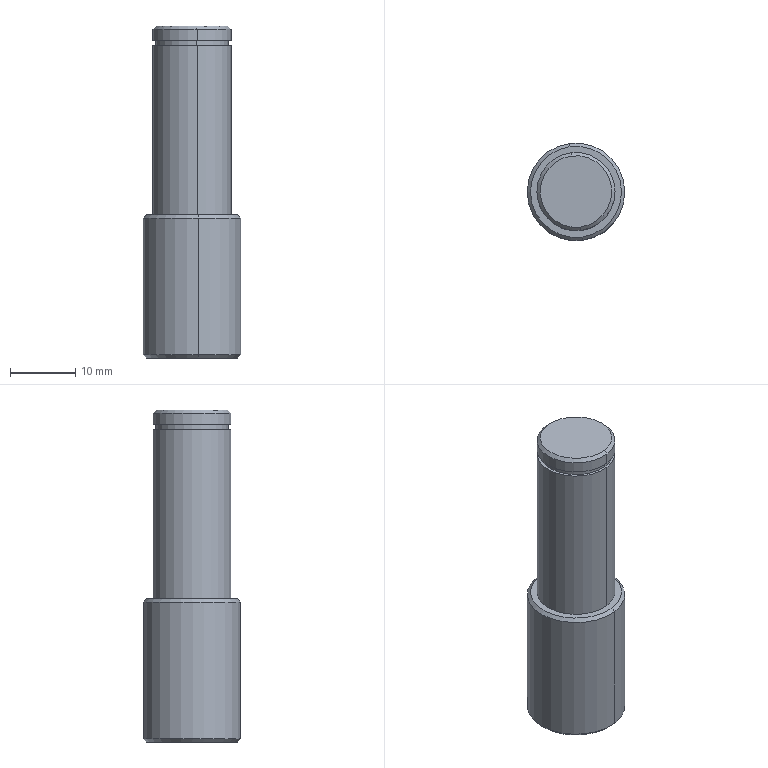Component | SolidWorks | DC-024-25-1 | 1 solid | 19 faces | box 15 x 15 x 51 mm | volume 7140 mm3 | cylinder 8 | cone 6 | plane 5 | commonest cylinder face diameters 12 x4 11.2 x2 15 x2
build123d program:
from build123d import *

# Parameters (mm, degrees)
SKETCH1_R           = 7.5
BOSS_EXTRUDE1_DEPTH = 22
SKETCH2_R           = 6
BOSS_EXTRUDE2_DEPTH = 29
SKETCH4_R           = 6
SKETCH4_R_2         = 5.6
CUT_EXTRUDE1_DEPTH  = 0.8
CHAMFER1_SIZE       = 0.5


with BuildPart() as part:
    # Sketch1 → Boss-Extrude1 (new body)
    with BuildSketch(Plane.XY):
        Circle(SKETCH1_R)
    extrude(amount=BOSS_EXTRUDE1_DEPTH)

    # Sketch2 → Boss-Extrude2 (add)
    with BuildSketch(Plane.XY.offset(22)):
        with Locations(Location((0, 0, 0), (0, 0, 180))):
            Circle(SKETCH2_R)
    extrude(amount=BOSS_EXTRUDE2_DEPTH)

    # Sketch4 → Cut-Extrude1 (cut)
    with BuildSketch(Plane.XY.offset(48)):
        with Locations(Location((0, 0, 0), (0, 0, 180))):
            Circle(SKETCH4_R)
        Circle(SKETCH4_R_2, mode=Mode.SUBTRACT)
    extrude(amount=CUT_EXTRUDE1_DEPTH, mode=Mode.SUBTRACT)

    # Chamfer1
    chamfer1_edges = [part.edges().sort_by_distance(p)[0] for p in [
        (-7.5, 0, 0),
        (-7.5, 0, 22),
        (6, 0, 51),
    ]]
    chamfer(chamfer1_edges, length=CHAMFER1_SIZE)


solid = part.part

# Placed as in the assembly
solid = solid.moved(Location((-25.633, 315.409, 3.5), (0, 0, 0)))
STEP:
#1=COLOUR_RGB('',0.7922,0.8196,0.9333);
#2=FILL_AREA_STYLE_COLOUR('',#1);
#3=FILL_AREA_STYLE('',(#2));
#4=SURFACE_STYLE_FILL_AREA(#3);
#5=SURFACE_SIDE_STYLE('',(#4));
#6=SURFACE_STYLE_USAGE(.BOTH.,#5);
#7=PRESENTATION_STYLE_ASSIGNMENT((#6));
#8=CARTESIAN_POINT('',(-0.9808,12.203,2.146));
#9=VERTEX_POINT('',#8);
#10=CARTESIAN_POINT('',(-1.038,12.632,2.146));
#11=VERTEX_POINT('',#10);
#12=CARTESIAN_POINT('',(-1.009,12.418,2.146));
#13=DIRECTION('',(0.,-0.,1.));
#14=DIRECTION('',(0.131,-0.9914,0.));
#15=AXIS2_PLACEMENT_3D('',#12,#13,#14);
#16=CIRCLE('',#15,0.2165);
#17=EDGE_CURVE('',#9,#11,#16,.T.);
#18=ORIENTED_EDGE('',*,*,#17,.F.);
#19=CARTESIAN_POINT('',(-0.9782,12.183,2.126));
#20=VERTEX_POINT('',#19);
#21=CARTESIAN_POINT('',(-0.9808,12.203,2.146));
#22=DIRECTION('',(0.09263,-0.701,-0.7071));
#23=VECTOR('',#22,39.37);
#24=LINE('',#21,#23);
#25=EDGE_CURVE('',#9,#20,#24,.T.);
#26=ORIENTED_EDGE('',*,*,#25,.T.);
#27=CARTESIAN_POINT('',(-1.04,12.652,2.126));
#28=VERTEX_POINT('',#27);
#29=CARTESIAN_POINT('',(-1.009,12.418,2.126));
#30=DIRECTION('',(-0.,0.,-1.));
#31=DIRECTION('',(0.131,-0.9914,0.));
#32=AXIS2_PLACEMENT_3D('',#29,#30,#31);
#33=CIRCLE('',#32,0.2362);
#34=EDGE_CURVE('',#28,#20,#33,.T.);
#35=ORIENTED_EDGE('',*,*,#34,.F.);
#36=CARTESIAN_POINT('',(-1.038,12.632,2.146));
#37=DIRECTION('',(-0.09263,0.701,-0.7071));
#38=VECTOR('',#37,39.37);
#39=LINE('',#36,#38);
#40=EDGE_CURVE('',#11,#28,#39,.T.);
#41=ORIENTED_EDGE('',*,*,#40,.F.);
#42=EDGE_LOOP('',(#18,#26,#35,#41));
#43=FACE_OUTER_BOUND('',#42,.T.);
#44=CARTESIAN_POINT('',(-1.009,12.418,2.146));
#45=DIRECTION('',(-0.,0.,-1.));
#46=DIRECTION('',(-0.131,0.9914,0.));
#47=AXIS2_PLACEMENT_3D('',#44,#45,#46);
#48=CONICAL_SURFACE('',#47,0.2165,0.7854);
#49=ADVANCED_FACE('',(#43),#48,.T.);
#50=CARTESIAN_POINT('',(-0.9731,12.144,1.004));
#51=VERTEX_POINT('',#50);
#52=CARTESIAN_POINT('',(-1.045,12.691,1.004));
#53=VERTEX_POINT('',#52);
#54=CARTESIAN_POINT('',(-1.009,12.418,1.004));
#55=DIRECTION('',(0.,-0.,1.));
#56=DIRECTION('',(0.131,-0.9914,0.));
#57=AXIS2_PLACEMENT_3D('',#54,#55,#56);
#58=CIRCLE('',#57,0.2756);
#59=EDGE_CURVE('',#51,#53,#58,.T.);
#60=ORIENTED_EDGE('',*,*,#59,.F.);
#61=CARTESIAN_POINT('',(-0.9705,12.125,0.9843));
#62=VERTEX_POINT('',#61);
#63=CARTESIAN_POINT('',(-0.9731,12.144,1.004));
#64=DIRECTION('',(0.09263,-0.701,-0.7071));
#65=VECTOR('',#64,39.37);
#66=LINE('',#63,#65);
#67=EDGE_CURVE('',#51,#62,#66,.T.);
#68=ORIENTED_EDGE('',*,*,#67,.T.);
#69=CARTESIAN_POINT('',(-1.048,12.71,0.9843));
#70=VERTEX_POINT('',#69);
#71=CARTESIAN_POINT('',(-1.009,12.418,0.9843));
#72=DIRECTION('',(-0.,0.,-1.));
#73=DIRECTION('',(0.131,-0.9914,0.));
#74=AXIS2_PLACEMENT_3D('',#71,#72,#73);
#75=CIRCLE('',#74,0.2953);
#76=EDGE_CURVE('',#70,#62,#75,.T.);
#77=ORIENTED_EDGE('',*,*,#76,.F.);
#78=CARTESIAN_POINT('',(-1.045,12.691,1.004));
#79=DIRECTION('',(-0.09263,0.701,-0.7071));
#80=VECTOR('',#79,39.37);
#81=LINE('',#78,#80);
#82=EDGE_CURVE('',#53,#70,#81,.T.);
#83=ORIENTED_EDGE('',*,*,#82,.F.);
#84=EDGE_LOOP('',(#60,#68,#77,#83));
#85=FACE_OUTER_BOUND('',#84,.T.);
#86=CARTESIAN_POINT('',(-1.009,12.418,1.004));
#87=DIRECTION('',(-0.,0.,-1.));
#88=DIRECTION('',(-0.131,0.9914,0.));
#89=AXIS2_PLACEMENT_3D('',#86,#87,#88);
#90=CONICAL_SURFACE('',#89,0.2756,0.7854);
#91=ADVANCED_FACE('',(#85),#90,.T.);
#92=CARTESIAN_POINT('',(-1.045,12.691,0.1378));
#93=VERTEX_POINT('',#92);
#94=CARTESIAN_POINT('',(-0.9731,12.144,0.1378));
#95=VERTEX_POINT('',#94);
#96=CARTESIAN_POINT('',(-1.009,12.418,0.1378));
#97=DIRECTION('',(-0.,0.,-1.));
#98=DIRECTION('',(0.131,-0.9914,0.));
#99=AXIS2_PLACEMENT_3D('',#96,#97,#98);
#100=CIRCLE('',#99,0.2756);
#101=EDGE_CURVE('',#93,#95,#100,.T.);
#102=ORIENTED_EDGE('',*,*,#101,.F.);
#103=CARTESIAN_POINT('',(-1.048,12.71,0.1575));
#104=VERTEX_POINT('',#103);
#105=CARTESIAN_POINT('',(-1.048,12.71,0.1575));
#106=DIRECTION('',(-0.09263,0.701,0.7071));
#107=VECTOR('',#106,39.37);
#108=LINE('',#105,#107);
#109=EDGE_CURVE('',#93,#104,#108,.T.);
#110=ORIENTED_EDGE('',*,*,#109,.T.);
#111=CARTESIAN_POINT('',(-0.9705,12.125,0.1575));
#112=VERTEX_POINT('',#111);
#113=CARTESIAN_POINT('',(-1.009,12.418,0.1575));
#114=DIRECTION('',(0.,-0.,1.));
#115=DIRECTION('',(0.131,-0.9914,0.));
#116=AXIS2_PLACEMENT_3D('',#113,#114,#115);
#117=CIRCLE('',#116,0.2953);
#118=EDGE_CURVE('',#112,#104,#117,.T.);
#119=ORIENTED_EDGE('',*,*,#118,.F.);
#120=CARTESIAN_POINT('',(-0.9705,12.125,0.1575));
#121=DIRECTION('',(0.09263,-0.701,0.7071));
#122=VECTOR('',#121,39.37);
#123=LINE('',#120,#122);
#124=EDGE_CURVE('',#95,#112,#123,.T.);
#125=ORIENTED_EDGE('',*,*,#124,.F.);
#126=EDGE_LOOP('',(#102,#110,#119,#125));
#127=FACE_OUTER_BOUND('',#126,.T.);
#128=CARTESIAN_POINT('',(-1.009,12.418,0.1575));
#129=DIRECTION('',(0.,-0.,1.));
#130=DIRECTION('',(0.131,-0.9914,0.));
#131=AXIS2_PLACEMENT_3D('',#128,#129,#130);
#132=CONICAL_SURFACE('',#131,0.2953,0.7854);
#133=ADVANCED_FACE('',(#127),#132,.T.);
#134=ORIENTED_EDGE('',*,*,#34,.T.);
#135=CARTESIAN_POINT('',(-0.9782,12.183,2.059));
#136=VERTEX_POINT('',#135);
#137=CARTESIAN_POINT('',(-0.9782,12.183,2.146));
#138=DIRECTION('',(-0.,0.,-1.));
#139=VECTOR('',#138,39.37);
#140=LINE('',#137,#139);
#141=EDGE_CURVE('',#20,#136,#140,.T.);
#142=ORIENTED_EDGE('',*,*,#141,.T.);
#143=CARTESIAN_POINT('',(-1.04,12.652,2.059));
#144=VERTEX_POINT('',#143);
#145=CARTESIAN_POINT('',(-1.009,12.418,2.059));
#146=DIRECTION('',(0.,-0.,1.));
#147=DIRECTION('',(0.131,-0.9914,0.));
#148=AXIS2_PLACEMENT_3D('',#145,#146,#147);
#149=CIRCLE('',#148,0.2362);
#150=EDGE_CURVE('',#136,#144,#149,.T.);
#151=ORIENTED_EDGE('',*,*,#150,.T.);
#152=CARTESIAN_POINT('',(-1.04,12.652,2.146));
#153=DIRECTION('',(-0.,0.,-1.));
#154=VECTOR('',#153,39.37);
#155=LINE('',#152,#154);
#156=EDGE_CURVE('',#28,#144,#155,.T.);
#157=ORIENTED_EDGE('',*,*,#156,.F.);
#158=EDGE_LOOP('',(#134,#142,#151,#157));
#159=FACE_OUTER_BOUND('',#158,.T.);
#160=CARTESIAN_POINT('',(-1.009,12.418,2.146));
#161=DIRECTION('',(-0.,0.,-1.));
#162=DIRECTION('',(-0.131,0.9914,0.));
#163=AXIS2_PLACEMENT_3D('',#160,#161,#162);
#164=CYLINDRICAL_SURFACE('',#163,0.2362);
#165=ADVANCED_FACE('',(#159),#164,.T.);
#166=CARTESIAN_POINT('',(-0.9803,12.199,2.059));
#167=VERTEX_POINT('',#166);
#168=CARTESIAN_POINT('',(-1.038,12.636,2.059));
#169=VERTEX_POINT('',#168);
#170=CARTESIAN_POINT('',(-1.009,12.418,2.059));
#171=DIRECTION('',(0.,-0.,1.));
#172=DIRECTION('',(0.131,-0.9914,0.));
#173=AXIS2_PLACEMENT_3D('',#170,#171,#172);
#174=CIRCLE('',#173,0.2205);
#175=EDGE_CURVE('',#167,#169,#174,.T.);
#176=ORIENTED_EDGE('',*,*,#175,.F.);
#177=CARTESIAN_POINT('',(-0.9803,12.199,2.028));
#178=VERTEX_POINT('',#177);
#179=CARTESIAN_POINT('',(-0.9803,12.199,2.059));
#180=DIRECTION('',(-0.,0.,-1.));
#181=VECTOR('',#180,39.37);
#182=LINE('',#179,#181);
#183=EDGE_CURVE('',#167,#178,#182,.T.);
#184=ORIENTED_EDGE('',*,*,#183,.T.);
#185=CARTESIAN_POINT('',(-1.038,12.636,2.028));
#186=VERTEX_POINT('',#185);
#187=CARTESIAN_POINT('',(-1.009,12.418,2.028));
#188=DIRECTION('',(0.,-0.,1.));
#189=DIRECTION('',(0.131,-0.9914,0.));
#190=AXIS2_PLACEMENT_3D('',#187,#188,#189);
#191=CIRCLE('',#190,0.2205);
#192=EDGE_CURVE('',#178,#186,#191,.T.);
#193=ORIENTED_EDGE('',*,*,#192,.T.);
#194=CARTESIAN_POINT('',(-1.038,12.636,2.059));
#195=DIRECTION('',(-0.,0.,-1.));
#196=VECTOR('',#195,39.37);
#197=LINE('',#194,#196);
#198=EDGE_CURVE('',#169,#186,#197,.T.);
#199=ORIENTED_EDGE('',*,*,#198,.F.);
#200=EDGE_LOOP('',(#176,#184,#193,#199));
#201=FACE_OUTER_BOUND('',#200,.T.);
#202=CARTESIAN_POINT('',(-1.009,12.418,2.059));
#203=DIRECTION('',(-0.,0.,-1.));
#204=DIRECTION('',(-0.131,0.9914,0.));
#205=AXIS2_PLACEMENT_3D('',#202,#203,#204);
#206=CYLINDRICAL_SURFACE('',#205,0.2205);
#207=ADVANCED_FACE('',(#201),#206,.T.);
#208=ORIENTED_EDGE('',*,*,#76,.T.);
#209=CARTESIAN_POINT('',(-0.9705,12.125,1.004));
#210=DIRECTION('',(-0.,0.,-1.));
#211=VECTOR('',#210,39.37);
#212=LINE('',#209,#211);
#213=EDGE_CURVE('',#62,#112,#212,.T.);
#214=ORIENTED_EDGE('',*,*,#213,.T.);
#215=ORIENTED_EDGE('',*,*,#118,.T.);
#216=CARTESIAN_POINT('',(-1.048,12.71,1.004));
#217=DIRECTION('',(-0.,0.,-1.));
#218=VECTOR('',#217,39.37);
#219=LINE('',#216,#218);
#220=EDGE_CURVE('',#70,#104,#219,.T.);
#221=ORIENTED_EDGE('',*,*,#220,.F.);
#222=EDGE_LOOP('',(#208,#214,#215,#221));
#223=FACE_OUTER_BOUND('',#222,.T.);
#224=CARTESIAN_POINT('',(-1.009,12.418,1.004));
#225=DIRECTION('',(-0.,0.,-1.));
#226=DIRECTION('',(-0.131,0.9914,0.));
#227=AXIS2_PLACEMENT_3D('',#224,#225,#226);
#228=CYLINDRICAL_SURFACE('',#227,0.2953);
#229=ADVANCED_FACE('',(#223),#228,.T.);
#230=CARTESIAN_POINT('',(-0.9782,12.183,2.028));
#231=VERTEX_POINT('',#230);
#232=CARTESIAN_POINT('',(-1.04,12.652,2.028));
#233=VERTEX_POINT('',#232);
#234=CARTESIAN_POINT('',(-1.009,12.418,2.028));
#235=DIRECTION('',(0.,-0.,1.));
#236=DIRECTION('',(0.131,-0.9914,0.));
#237=AXIS2_PLACEMENT_3D('',#234,#235,#236);
#238=CIRCLE('',#237,0.2362);
#239=EDGE_CURVE('',#231,#233,#238,.T.);
#240=ORIENTED_EDGE('',*,*,#239,.F.);
#241=CARTESIAN_POINT('',(-0.9782,12.183,1.004));
#242=VERTEX_POINT('',#241);
#243=CARTESIAN_POINT('',(-0.9782,12.183,2.146));
#244=DIRECTION('',(-0.,0.,-1.));
#245=VECTOR('',#244,39.37);
#246=LINE('',#243,#245);
#247=EDGE_CURVE('',#231,#242,#246,.T.);
#248=ORIENTED_EDGE('',*,*,#247,.T.);
#249=CARTESIAN_POINT('',(-1.04,12.652,1.004));
#250=VERTEX_POINT('',#249);
#251=CARTESIAN_POINT('',(-1.009,12.418,1.004));
#252=DIRECTION('',(0.,-0.,1.));
#253=DIRECTION('',(0.131,-0.9914,0.));
#254=AXIS2_PLACEMENT_3D('',#251,#252,#253);
#255=CIRCLE('',#254,0.2362);
#256=EDGE_CURVE('',#242,#250,#255,.T.);
#257=ORIENTED_EDGE('',*,*,#256,.T.);
#258=CARTESIAN_POINT('',(-1.04,12.652,2.146));
#259=DIRECTION('',(-0.,0.,-1.));
#260=VECTOR('',#259,39.37);
#261=LINE('',#258,#260);
#262=EDGE_CURVE('',#233,#250,#261,.T.);
#263=ORIENTED_EDGE('',*,*,#262,.F.);
#264=EDGE_LOOP('',(#240,#248,#257,#263));
#265=FACE_OUTER_BOUND('',#264,.T.);
#266=CARTESIAN_POINT('',(-1.009,12.418,2.146));
#267=DIRECTION('',(-0.,0.,-1.));
#268=DIRECTION('',(-0.131,0.9914,0.));
#269=AXIS2_PLACEMENT_3D('',#266,#267,#268);
#270=CYLINDRICAL_SURFACE('',#269,0.2362);
#271=ADVANCED_FACE('',(#265),#270,.T.);
#272=ORIENTED_EDGE('',*,*,#247,.F.);
#273=CARTESIAN_POINT('',(-1.009,12.418,2.028));
#274=DIRECTION('',(0.,-0.,1.));
#275=DIRECTION('',(0.131,-0.9914,0.));
#276=AXIS2_PLACEMENT_3D('',#273,#274,#275);
#277=CIRCLE('',#276,0.2362);
#278=EDGE_CURVE('',#233,#231,#277,.T.);
#279=ORIENTED_EDGE('',*,*,#278,.F.);
#280=ORIENTED_EDGE('',*,*,#262,.T.);
#281=CARTESIAN_POINT('',(-1.009,12.418,1.004));
#282=DIRECTION('',(0.,-0.,1.));
#283=DIRECTION('',(0.131,-0.9914,0.));
#284=AXIS2_PLACEMENT_3D('',#281,#282,#283);
#285=CIRCLE('',#284,0.2362);
#286=EDGE_CURVE('',#250,#242,#285,.T.);
#287=ORIENTED_EDGE('',*,*,#286,.T.);
#288=EDGE_LOOP('',(#272,#279,#280,#287));
#289=FACE_OUTER_BOUND('',#288,.T.);
#290=CARTESIAN_POINT('',(-1.009,12.418,2.146));
#291=DIRECTION('',(-0.,0.,-1.));
#292=DIRECTION('',(-0.131,0.9914,0.));
#293=AXIS2_PLACEMENT_3D('',#290,#291,#292);
#294=CYLINDRICAL_SURFACE('',#293,0.2362);
#295=ADVANCED_FACE('',(#289),#294,.T.);
#296=ORIENTED_EDGE('',*,*,#213,.F.);
#297=CARTESIAN_POINT('',(-1.009,12.418,0.9843));
#298=DIRECTION('',(-0.,0.,-1.));
#299=DIRECTION('',(0.131,-0.9914,0.));
#300=AXIS2_PLACEMENT_3D('',#297,#298,#299);
#301=CIRCLE('',#300,0.2953);
#302=EDGE_CURVE('',#62,#70,#301,.T.);
#303=ORIENTED_EDGE('',*,*,#302,.T.);
#304=ORIENTED_EDGE('',*,*,#220,.T.);
#305=CARTESIAN_POINT('',(-1.009,12.418,0.1575));
#306=DIRECTION('',(0.,-0.,1.));
#307=DIRECTION('',(0.131,-0.9914,0.));
#308=AXIS2_PLACEMENT_3D('',#305,#306,#307);
#309=CIRCLE('',#308,0.2953);
#310=EDGE_CURVE('',#104,#112,#309,.T.);
#311=ORIENTED_EDGE('',*,*,#310,.T.);
#312=EDGE_LOOP('',(#296,#303,#304,#311));
#313=FACE_OUTER_BOUND('',#312,.T.);
#314=CARTESIAN_POINT('',(-1.009,12.418,1.004));
#315=DIRECTION('',(-0.,0.,-1.));
#316=DIRECTION('',(-0.131,0.9914,0.));
#317=AXIS2_PLACEMENT_3D('',#314,#315,#316);
#318=CYLINDRICAL_SURFACE('',#317,0.2953);
#319=ADVANCED_FACE('',(#313),#318,.T.);
#320=CARTESIAN_POINT('',(-1.009,12.418,1.004));
#321=DIRECTION('',(0.,-0.,1.));
#322=DIRECTION('',(0.131,-0.9914,0.));
#323=AXIS2_PLACEMENT_3D('',#320,#321,#322);
#324=CIRCLE('',#323,0.2756);
#325=EDGE_CURVE('',#53,#51,#324,.T.);
#326=ORIENTED_EDGE('',*,*,#325,.T.);
#327=ORIENTED_EDGE('',*,*,#59,.T.);
#328=EDGE_LOOP('',(#326,#327));
#329=FACE_OUTER_BOUND('',#328,.T.);
#330=ORIENTED_EDGE('',*,*,#286,.F.);
#331=ORIENTED_EDGE('',*,*,#256,.F.);
#332=EDGE_LOOP('',(#330,#331));
#333=FACE_BOUND('',#332,.T.);
#334=CARTESIAN_POINT('',(-1.009,12.418,1.004));
#335=DIRECTION('',(-0.,-0.,1.));
#336=DIRECTION('',(0.131,-0.9914,-0.));
#337=AXIS2_PLACEMENT_3D('',#334,#335,#336);
#338=PLANE('',#337);
#339=ADVANCED_FACE('',(#329,#333),#338,.T.);
#340=CARTESIAN_POINT('',(-1.009,12.418,0.1378));
#341=DIRECTION('',(-0.,0.,-1.));
#342=DIRECTION('',(0.131,-0.9914,0.));
#343=AXIS2_PLACEMENT_3D('',#340,#341,#342);
#344=CIRCLE('',#343,0.2756);
#345=EDGE_CURVE('',#95,#93,#344,.T.);
#346=ORIENTED_EDGE('',*,*,#345,.T.);
#347=ORIENTED_EDGE('',*,*,#101,.T.);
#348=EDGE_LOOP('',(#346,#347));
#349=FACE_OUTER_BOUND('',#348,.T.);
#350=CARTESIAN_POINT('',(-1.009,12.418,0.1378));
#351=DIRECTION('',(-0.,-0.,1.));
#352=DIRECTION('',(0.131,-0.9914,-0.));
#353=AXIS2_PLACEMENT_3D('',#350,#351,#352);
#354=PLANE('',#353);
#355=ADVANCED_FACE('',(#349),#354,.F.);
#356=CARTESIAN_POINT('',(-1.009,12.418,2.059));
#357=DIRECTION('',(0.,-0.,1.));
#358=DIRECTION('',(0.131,-0.9914,0.));
#359=AXIS2_PLACEMENT_3D('',#356,#357,#358);
#360=CIRCLE('',#359,0.2362);
#361=EDGE_CURVE('',#144,#136,#360,.T.);
#362=ORIENTED_EDGE('',*,*,#361,.F.);
#363=ORIENTED_EDGE('',*,*,#150,.F.);
#364=EDGE_LOOP('',(#362,#363));
#365=FACE_OUTER_BOUND('',#364,.T.);
#366=CARTESIAN_POINT('',(-1.009,12.418,2.059));
#367=DIRECTION('',(0.,-0.,1.));
#368=DIRECTION('',(0.131,-0.9914,0.));
#369=AXIS2_PLACEMENT_3D('',#366,#367,#368);
#370=CIRCLE('',#369,0.2205);
#371=EDGE_CURVE('',#169,#167,#370,.T.);
#372=ORIENTED_EDGE('',*,*,#371,.T.);
#373=ORIENTED_EDGE('',*,*,#175,.T.);
#374=EDGE_LOOP('',(#372,#373));
#375=FACE_BOUND('',#374,.T.);
#376=CARTESIAN_POINT('',(-1.009,12.418,2.059));
#377=DIRECTION('',(-0.,-0.,1.));
#378=DIRECTION('',(0.131,-0.9914,-0.));
#379=AXIS2_PLACEMENT_3D('',#376,#377,#378);
#380=PLANE('',#379);
#381=ADVANCED_FACE('',(#365,#375),#380,.F.);
#382=ORIENTED_EDGE('',*,*,#278,.T.);
#383=ORIENTED_EDGE('',*,*,#239,.T.);
#384=EDGE_LOOP('',(#382,#383));
#385=FACE_OUTER_BOUND('',#384,.T.);
#386=CARTESIAN_POINT('',(-1.009,12.418,2.028));
#387=DIRECTION('',(0.,-0.,1.));
#388=DIRECTION('',(0.131,-0.9914,0.));
#389=AXIS2_PLACEMENT_3D('',#386,#387,#388);
#390=CIRCLE('',#389,0.2205);
#391=EDGE_CURVE('',#186,#178,#390,.T.);
#392=ORIENTED_EDGE('',*,*,#391,.F.);
#393=ORIENTED_EDGE('',*,*,#192,.F.);
#394=EDGE_LOOP('',(#392,#393));
#395=FACE_BOUND('',#394,.T.);
#396=CARTESIAN_POINT('',(-1.009,12.418,2.028));
#397=DIRECTION('',(-0.,-0.,1.));
#398=DIRECTION('',(0.131,-0.9914,-0.));
#399=AXIS2_PLACEMENT_3D('',#396,#397,#398);
#400=PLANE('',#399);
#401=ADVANCED_FACE('',(#385,#395),#400,.T.);
#402=ORIENTED_EDGE('',*,*,#183,.F.);
#403=ORIENTED_EDGE('',*,*,#371,.F.);
#404=ORIENTED_EDGE('',*,*,#198,.T.);
#405=ORIENTED_EDGE('',*,*,#391,.T.);
#406=EDGE_LOOP('',(#402,#403,#404,#405));
#407=FACE_OUTER_BOUND('',#406,.T.);
#408=CARTESIAN_POINT('',(-1.009,12.418,2.059));
#409=DIRECTION('',(-0.,0.,-1.));
#410=DIRECTION('',(-0.131,0.9914,0.));
#411=AXIS2_PLACEMENT_3D('',#408,#409,#410);
#412=CYLINDRICAL_SURFACE('',#411,0.2205);
#413=ADVANCED_FACE('',(#407),#412,.T.);
#414=CARTESIAN_POINT('',(-1.009,12.418,2.146));
#415=DIRECTION('',(0.,-0.,1.));
#416=DIRECTION('',(0.131,-0.9914,0.));
#417=AXIS2_PLACEMENT_3D('',#414,#415,#416);
#418=CIRCLE('',#417,0.2165);
#419=EDGE_CURVE('',#11,#9,#418,.T.);
#420=ORIENTED_EDGE('',*,*,#419,.T.);
#421=ORIENTED_EDGE('',*,*,#17,.T.);
#422=EDGE_LOOP('',(#420,#421));
#423=FACE_OUTER_BOUND('',#422,.T.);
#424=CARTESIAN_POINT('',(-1.009,12.418,2.146));
#425=DIRECTION('',(-0.,-0.,1.));
#426=DIRECTION('',(0.131,-0.9914,-0.));
#427=AXIS2_PLACEMENT_3D('',#424,#425,#426);
#428=PLANE('',#427);
#429=ADVANCED_FACE('',(#423),#428,.T.);
#430=ORIENTED_EDGE('',*,*,#141,.F.);
#431=CARTESIAN_POINT('',(-1.009,12.418,2.126));
#432=DIRECTION('',(-0.,0.,-1.));
#433=DIRECTION('',(0.131,-0.9914,0.));
#434=AXIS2_PLACEMENT_3D('',#431,#432,#433);
#435=CIRCLE('',#434,0.2362);
#436=EDGE_CURVE('',#20,#28,#435,.T.);
#437=ORIENTED_EDGE('',*,*,#436,.T.);
#438=ORIENTED_EDGE('',*,*,#156,.T.);
#439=ORIENTED_EDGE('',*,*,#361,.T.);
#440=EDGE_LOOP('',(#430,#437,#438,#439));
#441=FACE_OUTER_BOUND('',#440,.T.);
#442=CARTESIAN_POINT('',(-1.009,12.418,2.146));
#443=DIRECTION('',(-0.,0.,-1.));
#444=DIRECTION('',(-0.131,0.9914,0.));
#445=AXIS2_PLACEMENT_3D('',#442,#443,#444);
#446=CYLINDRICAL_SURFACE('',#445,0.2362);
#447=ADVANCED_FACE('',(#441),#446,.T.);
#448=ORIENTED_EDGE('',*,*,#109,.F.);
#449=ORIENTED_EDGE('',*,*,#345,.F.);
#450=ORIENTED_EDGE('',*,*,#124,.T.);
#451=ORIENTED_EDGE('',*,*,#310,.F.);
#452=EDGE_LOOP('',(#448,#449,#450,#451));
#453=FACE_OUTER_BOUND('',#452,.T.);
#454=CARTESIAN_POINT('',(-1.009,12.418,0.1575));
#455=DIRECTION('',(0.,-0.,1.));
#456=DIRECTION('',(0.131,-0.9914,0.));
#457=AXIS2_PLACEMENT_3D('',#454,#455,#456);
#458=CONICAL_SURFACE('',#457,0.2953,0.7854);
#459=ADVANCED_FACE('',(#453),#458,.T.);
#460=ORIENTED_EDGE('',*,*,#67,.F.);
#461=ORIENTED_EDGE('',*,*,#325,.F.);
#462=ORIENTED_EDGE('',*,*,#82,.T.);
#463=ORIENTED_EDGE('',*,*,#302,.F.);
#464=EDGE_LOOP('',(#460,#461,#462,#463));
#465=FACE_OUTER_BOUND('',#464,.T.);
#466=CARTESIAN_POINT('',(-1.009,12.418,1.004));
#467=DIRECTION('',(-0.,0.,-1.));
#468=DIRECTION('',(-0.131,0.9914,0.));
#469=AXIS2_PLACEMENT_3D('',#466,#467,#468);
#470=CONICAL_SURFACE('',#469,0.2756,0.7854);
#471=ADVANCED_FACE('',(#465),#470,.T.);
#472=ORIENTED_EDGE('',*,*,#25,.F.);
#473=ORIENTED_EDGE('',*,*,#419,.F.);
#474=ORIENTED_EDGE('',*,*,#40,.T.);
#475=ORIENTED_EDGE('',*,*,#436,.F.);
#476=EDGE_LOOP('',(#472,#473,#474,#475));
#477=FACE_OUTER_BOUND('',#476,.T.);
#478=CARTESIAN_POINT('',(-1.009,12.418,2.146));
#479=DIRECTION('',(-0.,0.,-1.));
#480=DIRECTION('',(-0.131,0.9914,0.));
#481=AXIS2_PLACEMENT_3D('',#478,#479,#480);
#482=CONICAL_SURFACE('',#481,0.2165,0.7854);
#483=ADVANCED_FACE('',(#477),#482,.T.);
#484=CLOSED_SHELL('',(#49,#91,#133,#165,#207,#229,#271,#295,#319,#339,#355,#381,#401,#413,#429,#447,#459,#471,#483));
#485=MANIFOLD_SOLID_BREP('',#484);
#486=STYLED_ITEM('',(#7),#485);
#487=(LENGTH_UNIT()NAMED_UNIT(*)SI_UNIT($,.METRE.));
#488=LENGTH_MEASURE_WITH_UNIT(LENGTH_MEASURE(0.0254),#487);
#489=DIMENSIONAL_EXPONENTS(1.,0.,0.,0.,0.,0.,0.);
#490=(CONVERSION_BASED_UNIT('',#488)LENGTH_UNIT()NAMED_UNIT(#489));
#491=UNCERTAINTY_MEASURE_WITH_UNIT(LENGTH_MEASURE(0.00001),#490,'','');
#492=(NAMED_UNIT(*)PLANE_ANGLE_UNIT()SI_UNIT($,.RADIAN.));
#493=(NAMED_UNIT(*)SI_UNIT($,.STERADIAN.)SOLID_ANGLE_UNIT());
#494=(GEOMETRIC_REPRESENTATION_CONTEXT(3)GLOBAL_UNCERTAINTY_ASSIGNED_CONTEXT((#491))GLOBAL_UNIT_ASSIGNED_CONTEXT((#490,#492,#493))REPRESENTATION_CONTEXT('',''));
#495=MECHANICAL_DESIGN_GEOMETRIC_PRESENTATION_REPRESENTATION('',(#486),#494);
#496=PRESENTATION_LAYER_ASSIGNMENT('','',(#486));
#497=CARTESIAN_POINT('',(0.,0.,0.));
#498=DIRECTION('',(0.,0.,1.));
#499=DIRECTION('',(1.,0.,0.));
#500=AXIS2_PLACEMENT_3D('',#497,#498,#499);
#501=(LENGTH_UNIT()NAMED_UNIT(*)SI_UNIT($,.METRE.));
#502=LENGTH_MEASURE_WITH_UNIT(LENGTH_MEASURE(0.0254),#501);
#503=DIMENSIONAL_EXPONENTS(1.,0.,0.,0.,0.,0.,0.);
#504=(CONVERSION_BASED_UNIT('',#502)LENGTH_UNIT()NAMED_UNIT(#503));
#505=UNCERTAINTY_MEASURE_WITH_UNIT(LENGTH_MEASURE(0.00001),#504,'','');
#506=(NAMED_UNIT(*)PLANE_ANGLE_UNIT()SI_UNIT($,.RADIAN.));
#507=(NAMED_UNIT(*)SI_UNIT($,.STERADIAN.)SOLID_ANGLE_UNIT());
#508=(GEOMETRIC_REPRESENTATION_CONTEXT(3)GLOBAL_UNCERTAINTY_ASSIGNED_CONTEXT((#505))GLOBAL_UNIT_ASSIGNED_CONTEXT((#504,#506,#507))REPRESENTATION_CONTEXT('',''));
#509=ADVANCED_BREP_SHAPE_REPRESENTATION('',(#485,#500),#508);